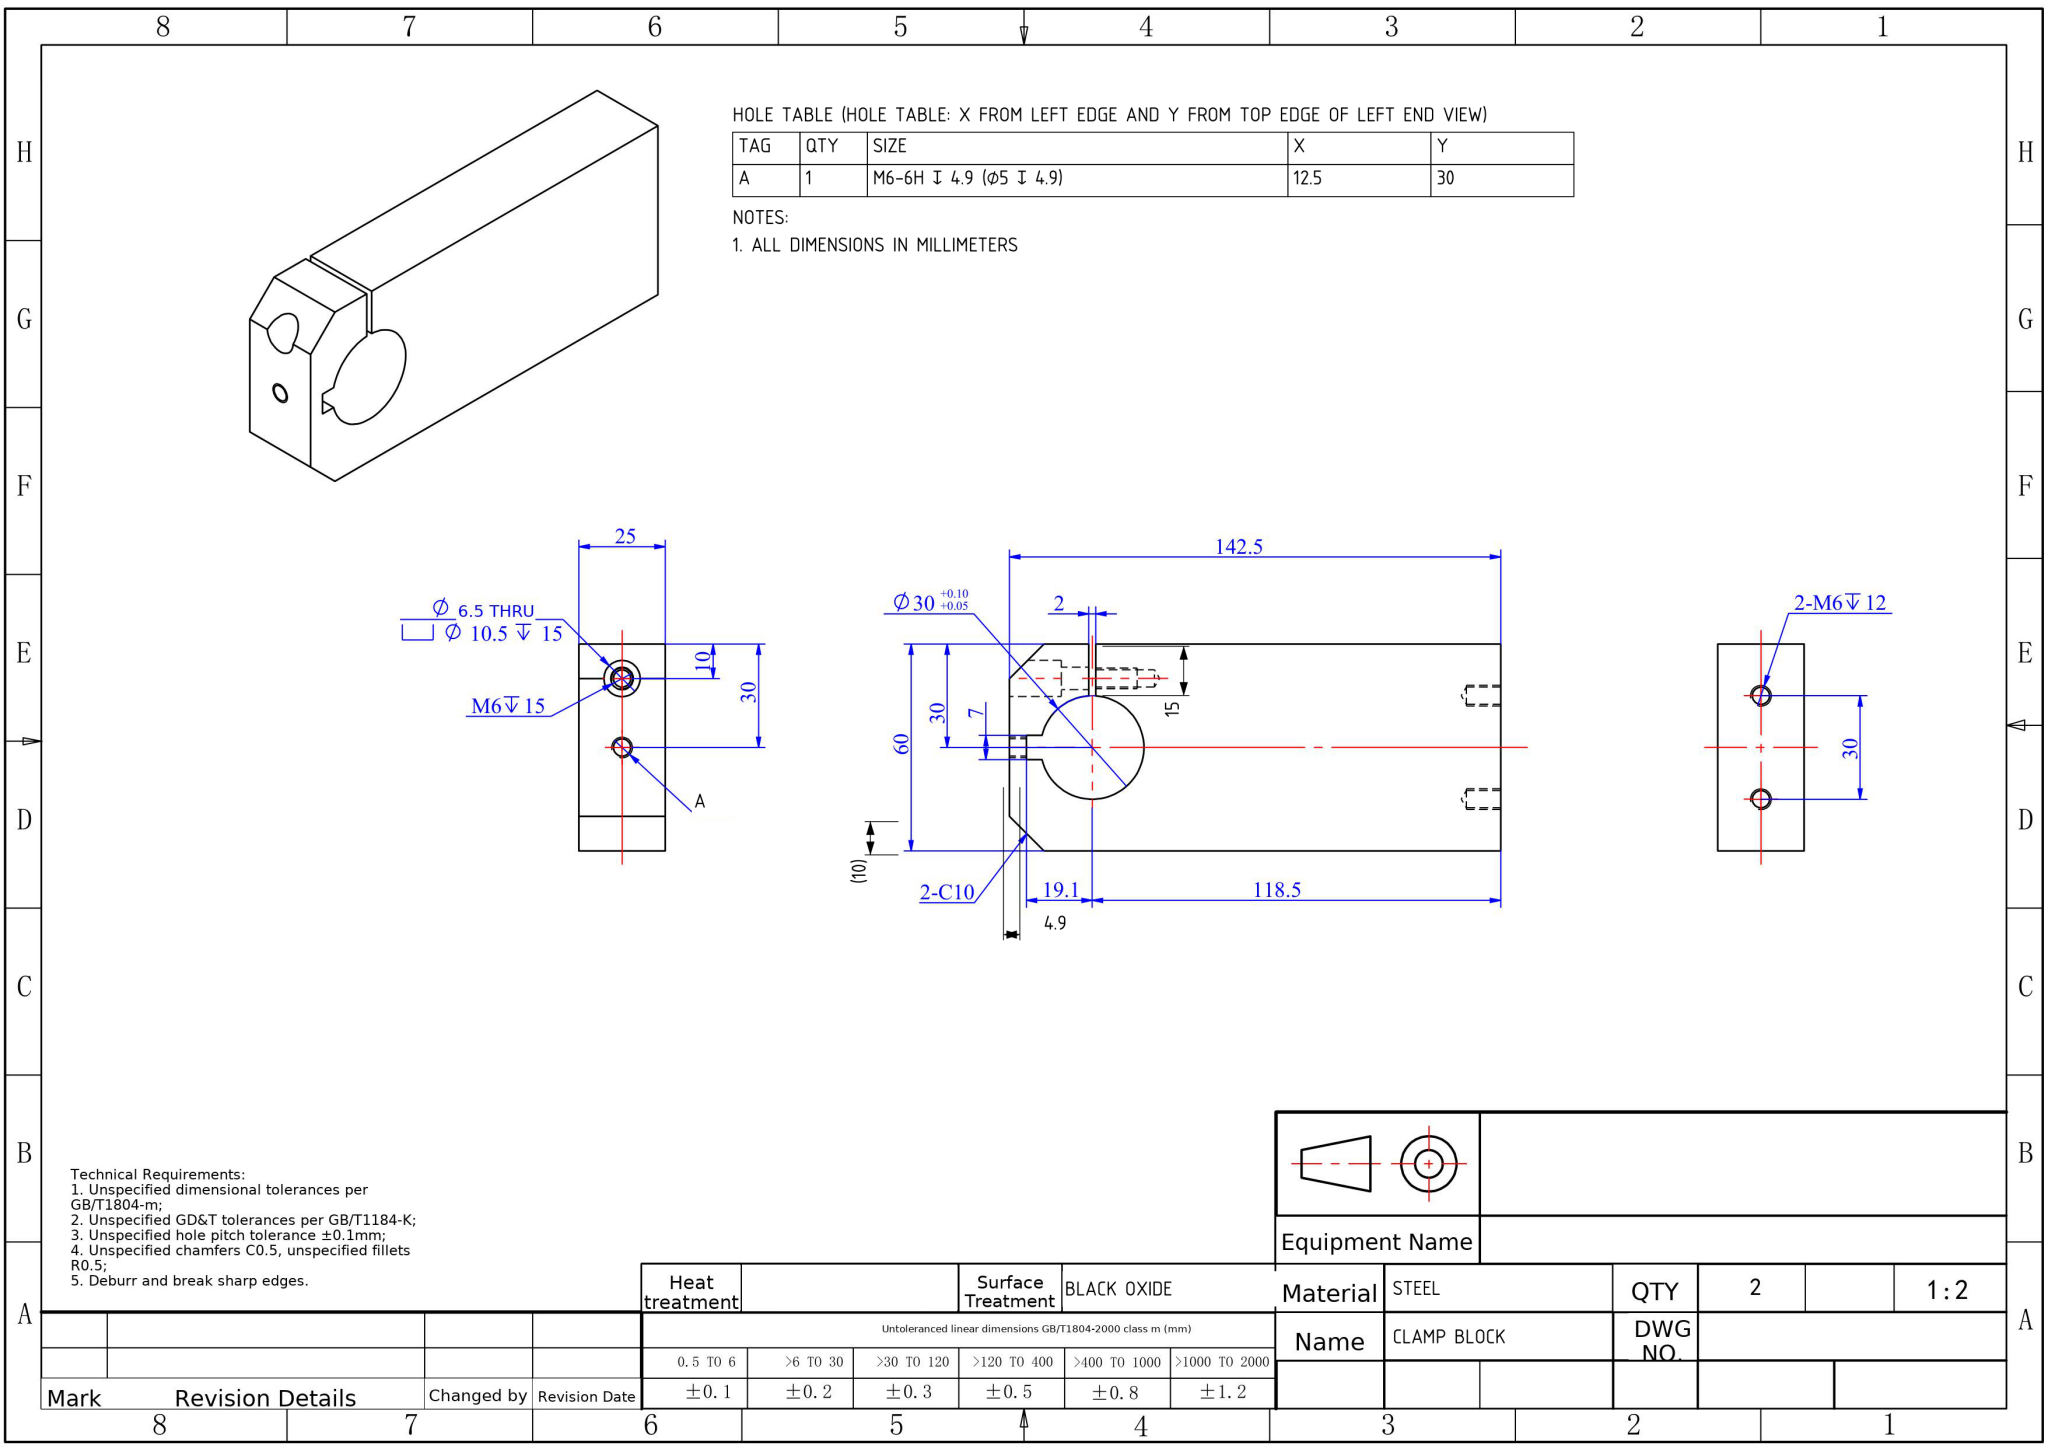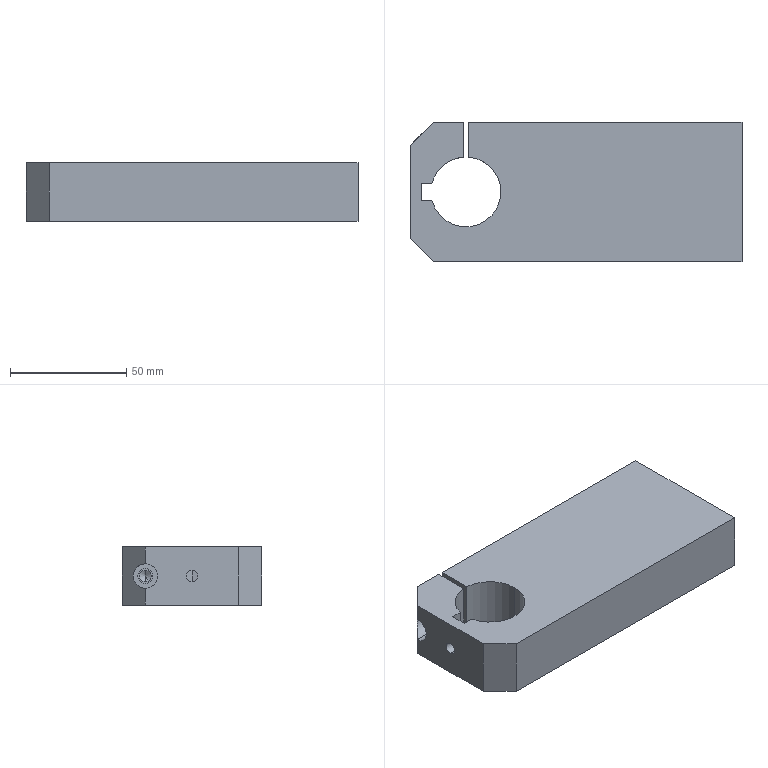Part | NX | mm | 1 solid | 36 faces | box 142.5 x 60 x 25 mm | volume 189766 mm3 | cylinder 15 | plane 15 | cone 6 | commonest cylinder face diameters 5 x8 30 x3 10.5 x2 6.5 x2